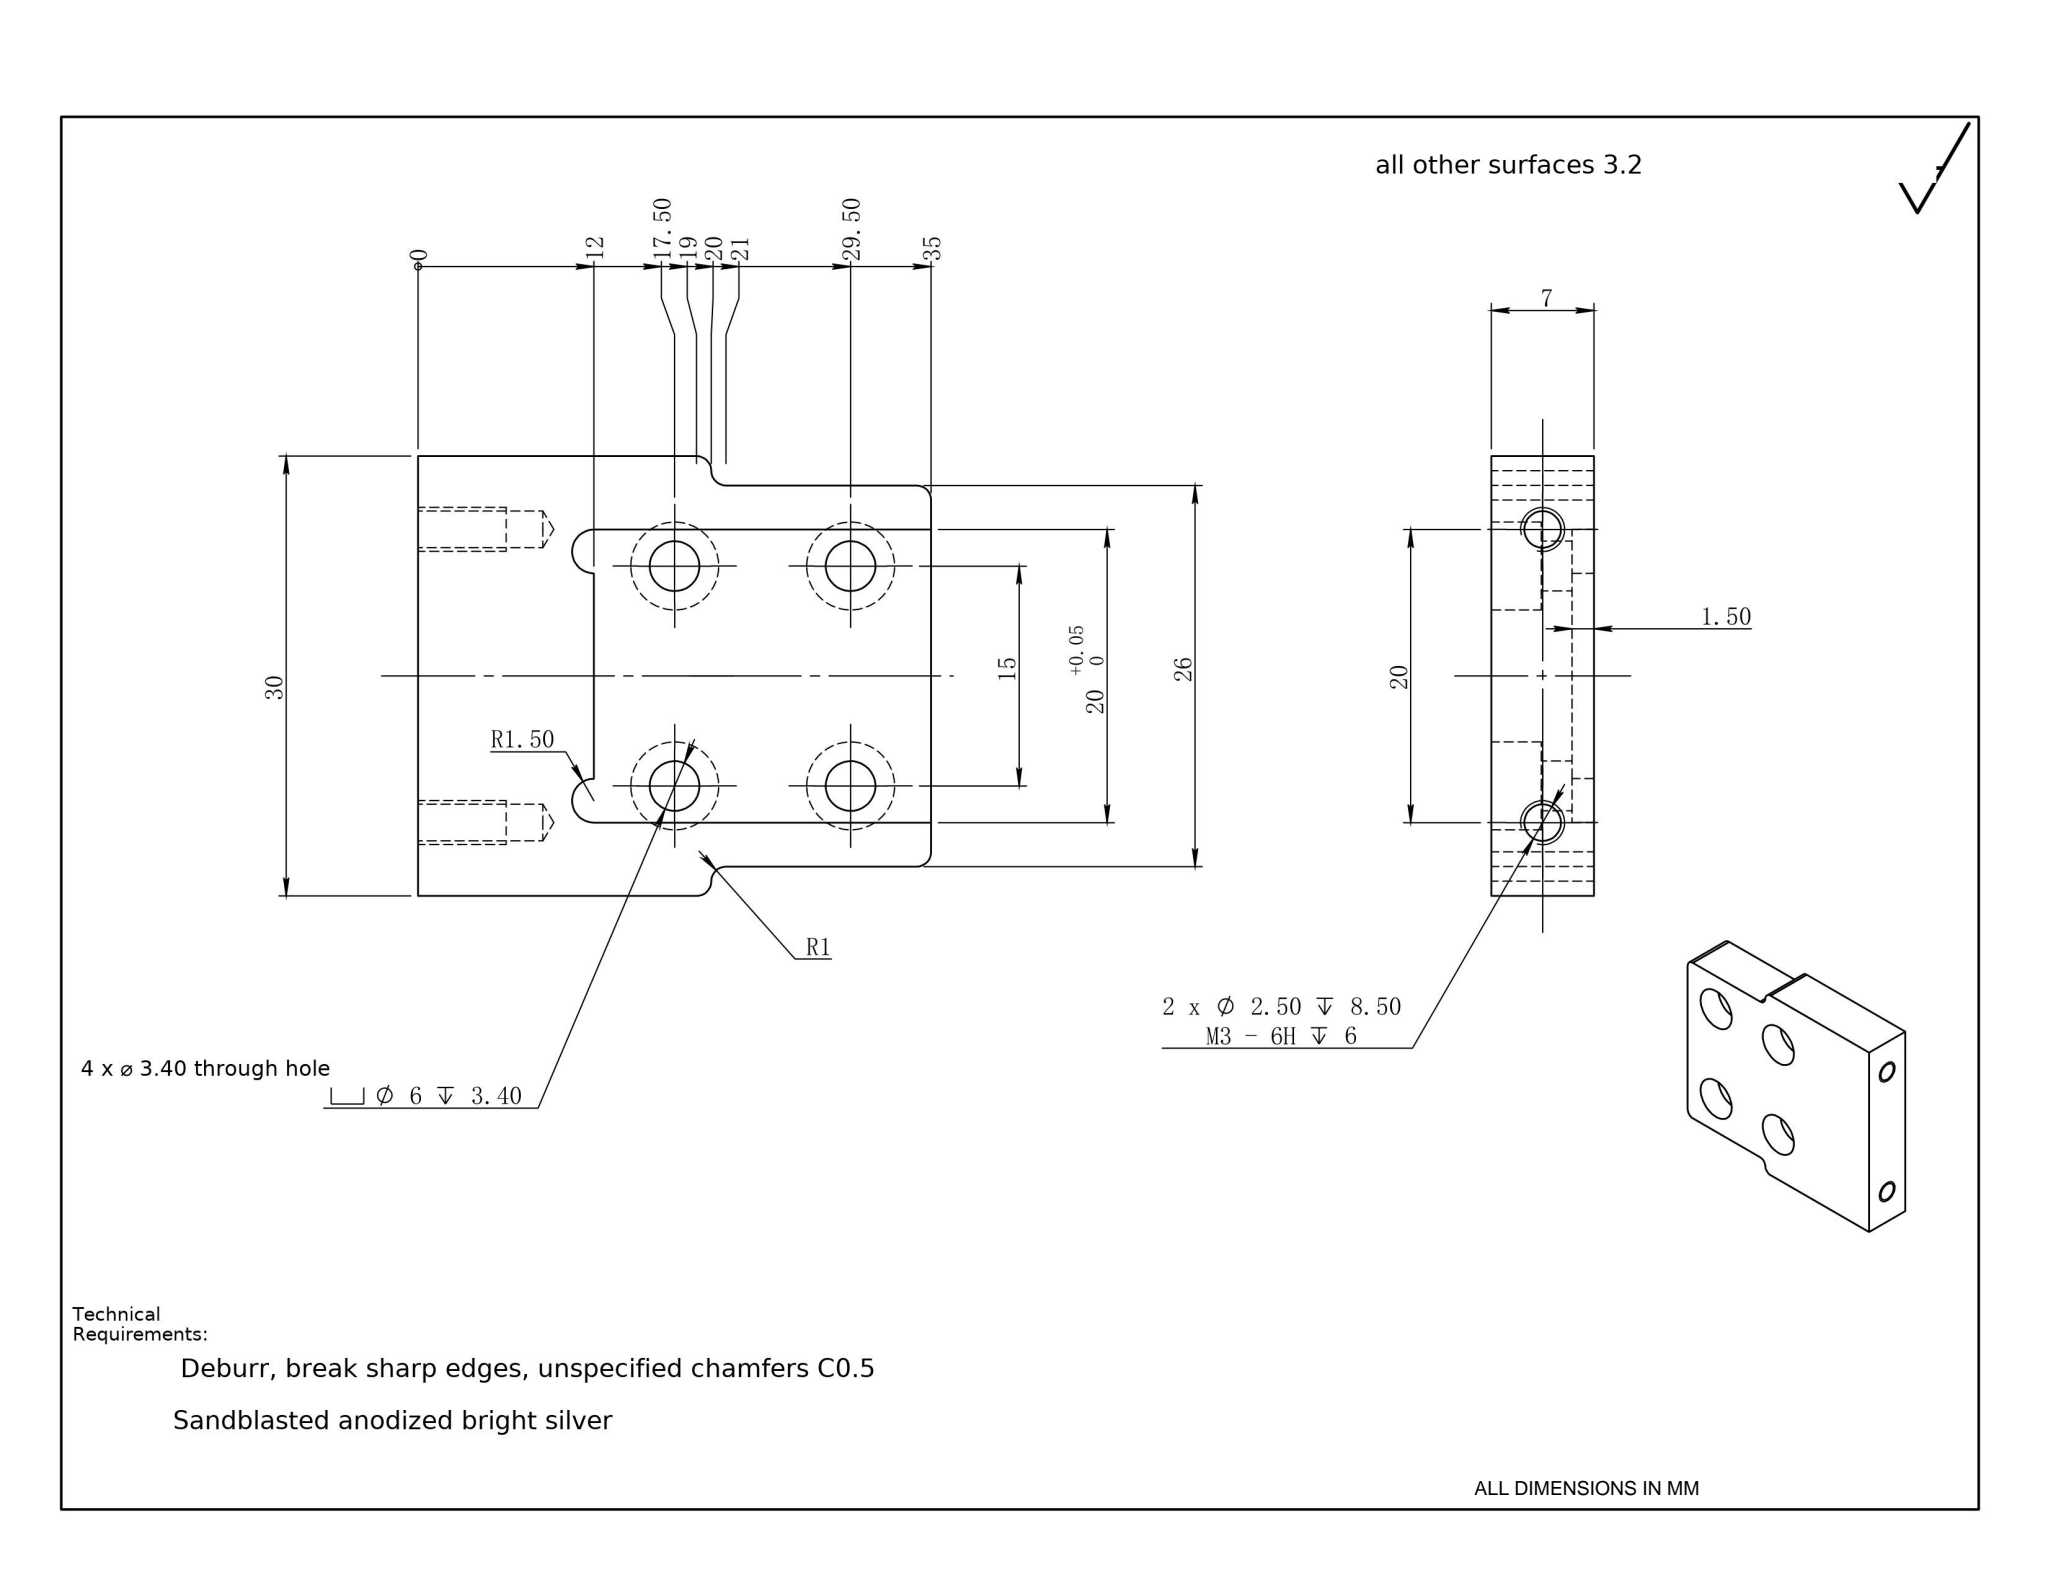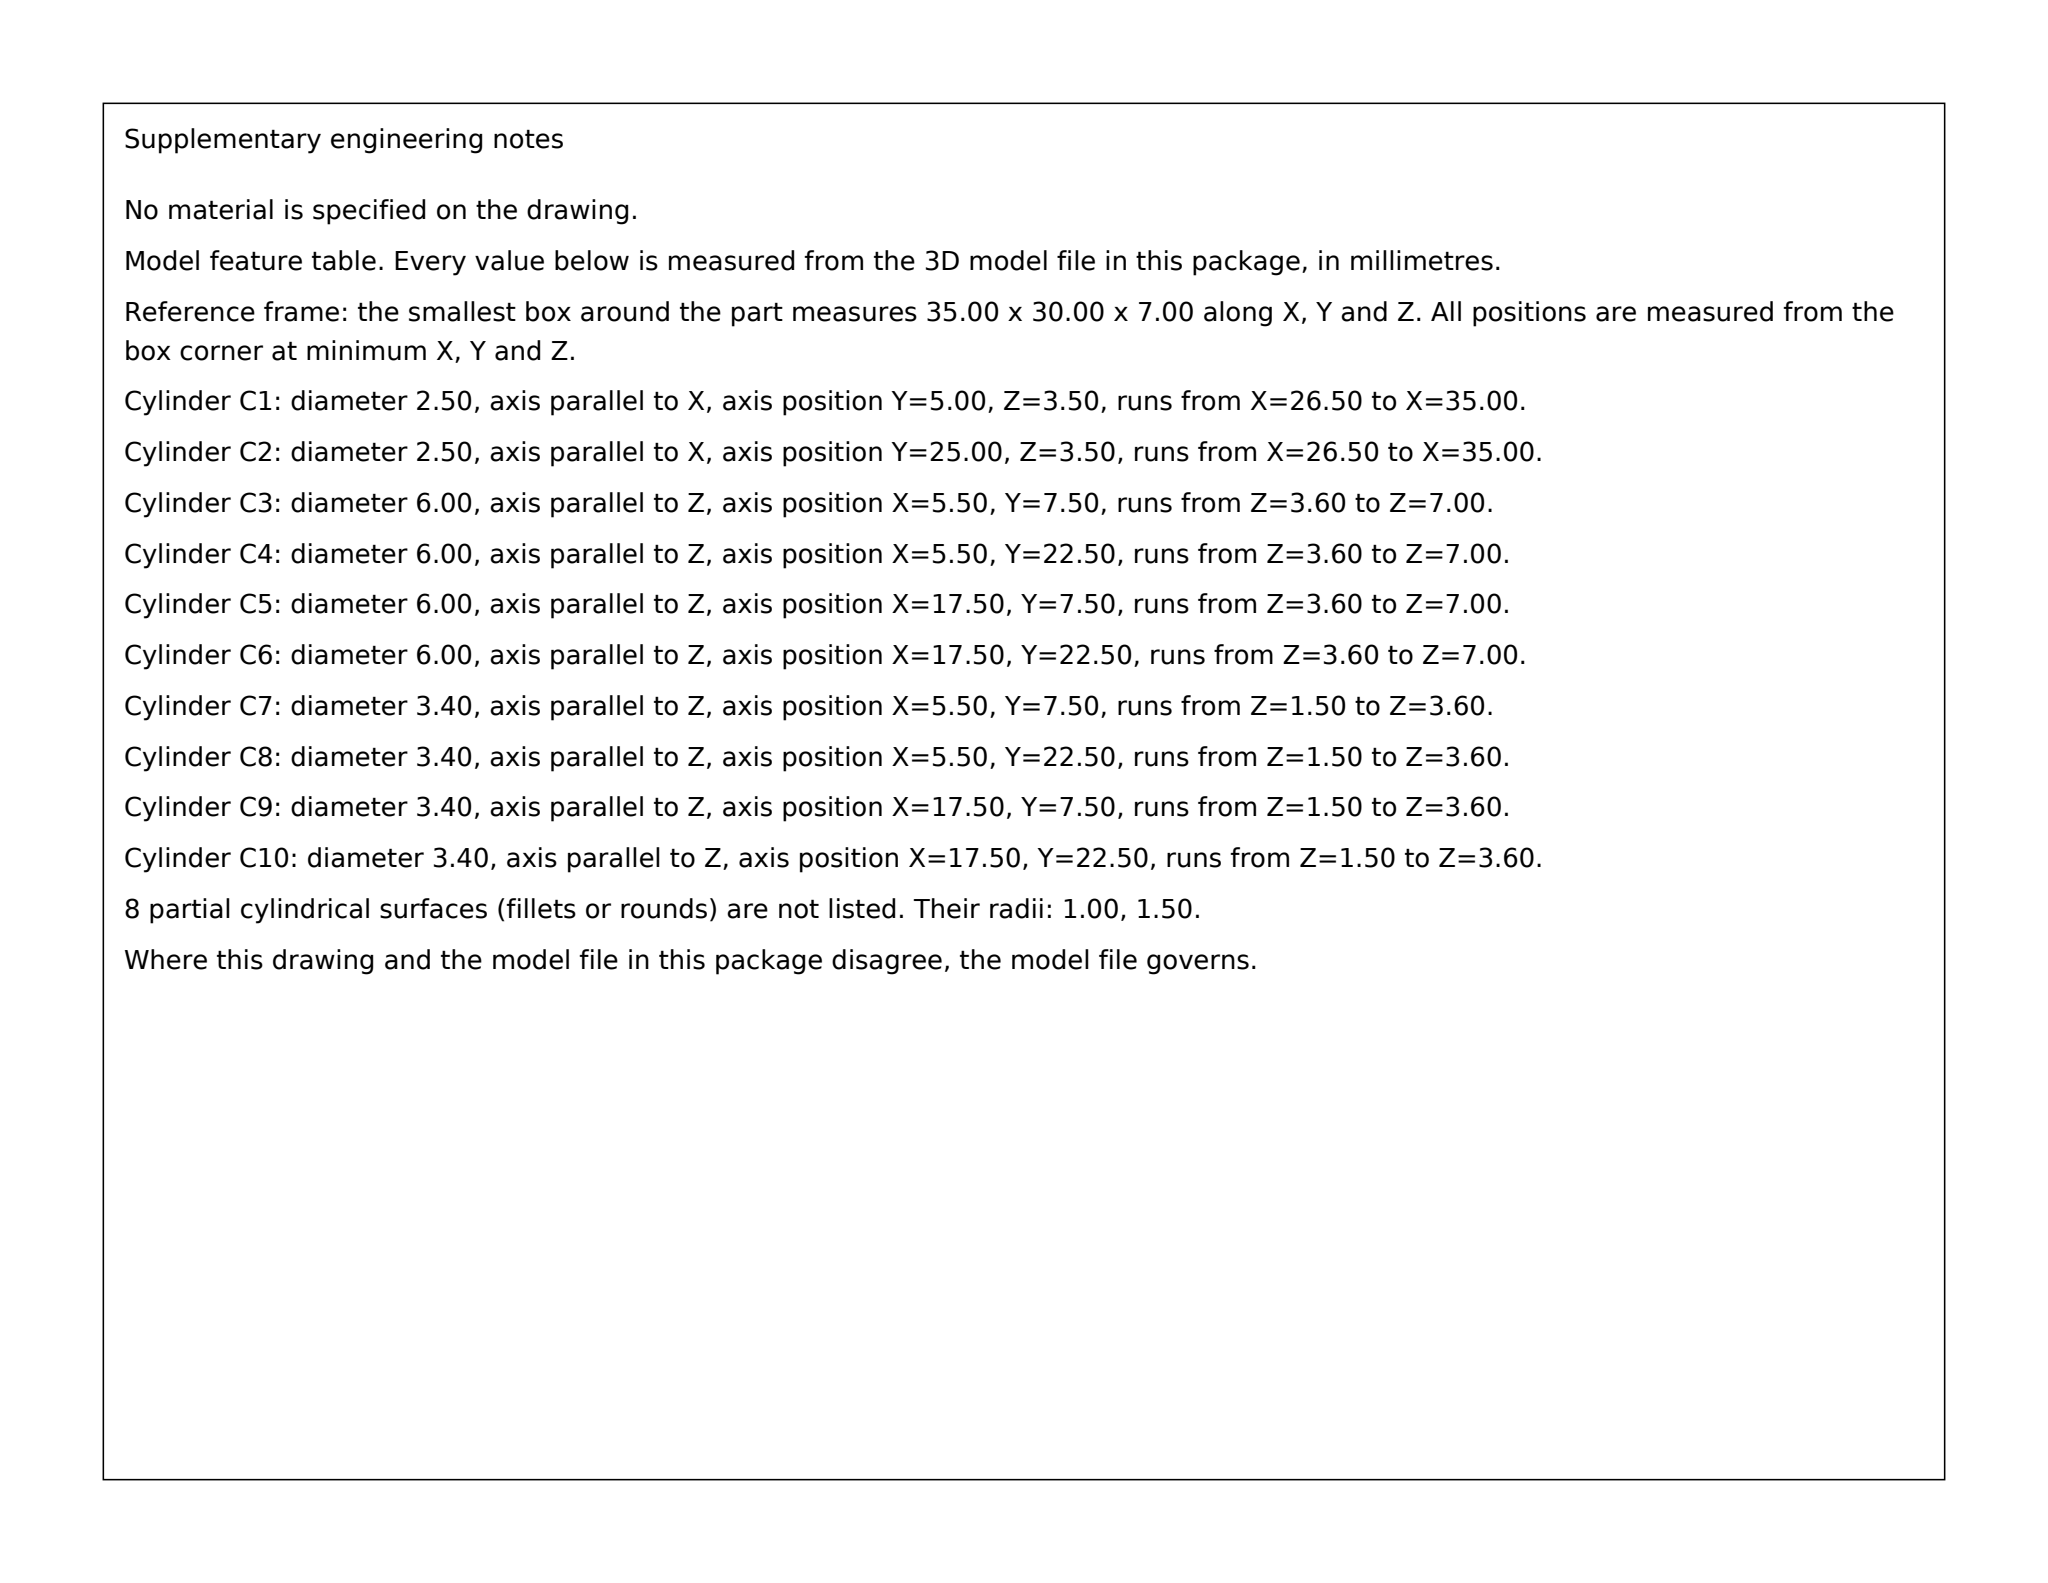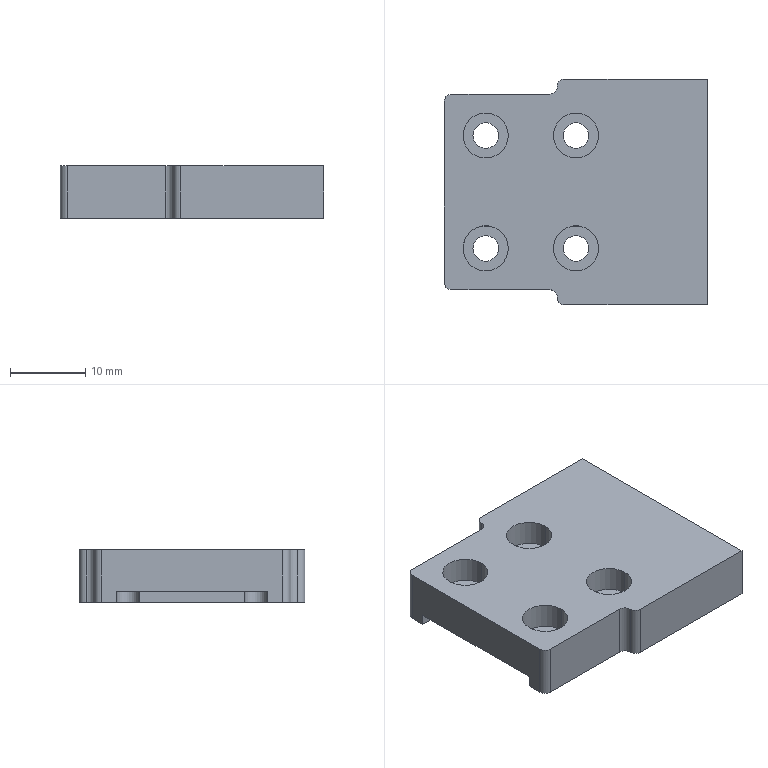Part | SolidWorks | mm | 1 solid | 48 faces | box 35 x 30 x 7 mm | volume 5680 mm3 | cylinder 28 | plane 16 | cone 4 | commonest cylinder face diameters 6 x8 3.4 x8 2 x6 2.5 x4 3 x2